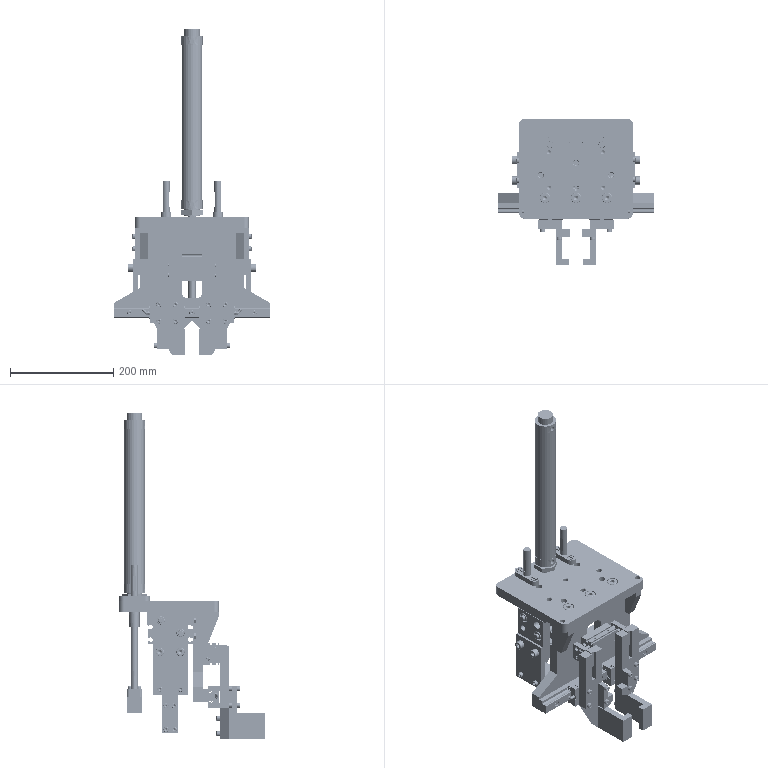Assembly | NX | mm | 90 component files | 90 solids | 2789 faces | box 300 x 282.7 x 629.92 mm | volume 4094625 mm3 | plane 1543 | cone 552 | cylinder 475 | spline 109 | torus 108 | sphere 2 | commonest cylinder face diameters 6 x76 5 x65 10 x55 8 x34 3.5 x28 20 x23 4.2 x18 6.6 x17
Bill of materials:
unnamed part 1 | 2 |  | Flanged post: a flat obround (slot-shaped) flange with a cylindrical post perpendicular to it at the center. A central bore runs down through the post, and there is a counterbored hole near each rounded end of the flange.
unnamed part 2 | 4 |  | Slotted cheese-style screw: a cylindrical head with slightly tapered sides and a straight slot across the top, a short plain neck, and an externally threaded shank.
unnamed part 3 | 2 |  | Rectangular block with a stepped notch along one lower edge. It has several round through holes of different sizes, and two cylindrical pins pass through it, sticking out a long way on one face and a short way on the other.
unnamed part 4 | 2 |  | Angled fitting-like body: a straight cylindrical section with a hex band partway along it, joined by a rounded bend to a shorter angled section. The angled section has a hex collar and a tapered, faceted end.
unnamed part 5 | 12 |  | Socket head cap screw style fastener: a cylindrical head with a hexagonal socket recess on top and a long, fully threaded shank.
unnamed part 6 | 1 |  | Rectangular prismatic block. One long face has two parallel lengthwise grooves with two drilled holes between them. An end face has four large round holes and four edge notches with rounded bottoms, and the side faces have smaller holes.
unnamed part 7 | 2 |  | Slender cylindrical pin or rod with a short reduced-diameter neck (groove) near one end. A possible small flat or surface feature is also visible near that end.
unnamed part 8 | 5 |  | Short socket head cap screw style fastener: a cylindrical head with a hexagonal socket and a threaded shank about one and a half head lengths long.
unnamed part 9 | 2 |  | L-shaped block of constant thickness: a tall rectangular leg and a shorter, wider foot portion with an angled cut at its bottom. Two round through holes are spaced along the tall leg.
unnamed part 10 | 4 |  | Hex head bolt style fastener: a hexagonal head with chamfered corners and a threaded shank running almost to the head.
unnamed part 11 | 2 |  | Thin rectangular plate with four round through holes near the corners: two larger holes at one end and two smaller at the other. There is a shallow rectangular groove or step across one face near the small-hole end.
unnamed part 12 | 2 |  | Bracket of two flat plates joined at a right angle: a solid rectangular top plate and a narrower vertical web, flush with one edge of the top plate, with four round through holes in a 2x2 pattern. It looks T-shaped from one side and L-shaped from the other.
unnamed part 13 | 4 |  | Long socket-head cap screw: a cylindrical head with a hexagonal socket recess on a long, fully threaded slender shank.
unnamed part 14 | 2 |  | Flat bar plate with a straight open-ended slot cut in from one end, a tapered (angled) edge at the opposite end, and a pattern of small through-holes.
unnamed part 15 | 3 |  | Rectangular block with a V-shaped notch cut across one face, leaving two lugs, each with two through-holes.
unnamed part 16 | 2 |  | Rectangular plate with a stepped edge, with two parallel cylindrical rods pressed through it. The rods stick out a short way on one side and a long way on the other. The plate also has extra holes.
unnamed part 17 | 4 |  | Short socket-head-style cap screw with a cylindrical head and a fully threaded shank.
unnamed part 18 | 4 |  | Thin rectangular plate with a large C-shaped cutout on one long edge. The cutout has lobed/notched corners, and the plate carries raised or recessed features, including two small counterbored hex-shaped holes.
unnamed part 19 | 1 |  | Upright rectangular plate on a wider base flange with angled gussets at both sides. It has a central rounded-rectangle through-slot and several hole patterns.
unnamed part 20 | 2 |  | Solid prismatic wedge block: rectangular in two views, with one face tapered at an angle along most of its height.
unnamed part 21 | 2 |  | Rectangular block with a C-shaped channel profile running its full length. The middle body is slightly larger than the end sections, and there are mounting holes on the top and side faces.
unnamed part 22 | 1 |  | Flat rectangular plate with rounded corners, many through-holes of several sizes (some counterbored), and a small rectangular notch on one edge underside.
unnamed part 23 | 4 |  | Socket-head cap screw with a cylindrical head, a hexagonal socket and a fully threaded shank of moderate length.
unnamed part 24 | 2 |  | L-section rectangular bar or block: a thin plate with a short perpendicular foot along one edge, extruded with a constant profile.
unnamed part 25 | 4 |  | Socket head cap screw-like fastener: cylindrical head with hexagonal socket, long fully threaded shank.
unnamed part 26 | 1 |  | Rectangular bar/plate with rounded corners and a symmetric pattern of holes: two larger holes near the ends, a larger central through hole, and four smaller through holes around the center.
unnamed part 27 | 1 |  | Long straight prismatic rail with a constant profile featuring longitudinal grooves on the side faces and a row of five evenly spaced holes along its length.
unnamed part 28 | 4 |  | Socket head cap screw-like fastener with cylindrical head, hexagonal socket and a threaded shank of moderate length.
unnamed part 29 | 1 |  | Slender elongated cylindrical body with end caps, a smaller-diameter rod extending from one end, and a hexagonal flange/collar feature near the rod end.
unnamed part 30 | 4 |  | Cap-screw-like fastener with a plain cylindrical head and a long threaded shank.
unnamed part 31 | 1 |  | Rectangular block with longitudinal grooves along two opposite sides, a shallow large circular recess and multiple small holes on the top face, through holes on the end faces, and semicircular edge notches.
unnamed part 32 | 3 |  | Short socket head cap screw-like fastener: cylindrical head with hexagonal socket and a short threaded shank.
Mates:
1. touch align | Cyl_Fix_Plate 1 face | Cyl_Fix_Vert_Plate 1 face
2. concentric | Cyl_Fix_Vert_Plate 1 edge | Cyl_Fix_Plate 1 edge
3. concentric | V_Block 3 edge | V_Block_Fix_Plate 1 edge
4. concentric | V_Block 3 edge | V_Block_Fix_Plate 1 edge
5. concentric | Reinforce_Rib 1 edge | Cyl_Fix_Vert_Plate 1 edge
6. concentric | Reinforce_Rib 2 edge | Cyl_Fix_Vert_Plate 1 edge
7. concentric | Reinforce_Rib 2 edge | Cyl_Fix_Vert_Plate 1 edge
8. concentric | Reinforce_Rib 1 edge | Cyl_Fix_Vert_Plate 1 edge
9. concentric | Column_Cyl 1 edge | V_Block_Fix_Plate 1 edge
10. concentric | Guide_Rod 1 edge | V_Block_Fix_Plate 1 edge
11. concentric | Guide_Rod 2 edge | V_Block_Fix_Plate 1 edge
12. concentric | Guide_Bush 2 edge | Cyl_Fix_Plate 1 edge
13. concentric | Guide_Bush 2 edge | Cyl_Fix_Plate 1 edge
14. concentric | Guide_Bush 1 edge | Cyl_Fix_Plate 1 edge
15. concentric | Guide_Bush 1 edge | Cyl_Fix_Plate 1 edge
16. concentric | Clamp_Cyl_1 1 edge | Cyl_Fix_Vert_Plate 1 edge
17. concentric | Clamp_Cyl_1 1 edge | Cyl_Fix_Vert_Plate 1 edge
18. concentric | Nylon_Stopper_Block 1 edge | Aux_Gripper_Jaw_Vert_Plate 1 edge
19. concentric | Nylon_Stopper_Block 2 edge | Aux_Gripper_Jaw_Vert_Plate 2 edge
20. concentric | Nylon_Stopper_Block 1 edge | Aux_Gripper_Jaw_Vert_Plate 1 edge
21. concentric | Nylon_Stopper_Block 2 edge | Aux_Gripper_Jaw_Vert_Plate 2 edge
22. fit | Guide_Rod 2 face | Guide_Bush 2 edge
23. fit | Guide_Rod 1 face | Guide_Bush 1 face
24. fit | Aux_Clamp_Cyl_Comp 1 face | Clamp_Cyl_1 1 edge
25. fit | Aux_Clamp_Cyl_Comp 2 face | Clamp_Cyl_1 1 edge
26. fit | Aux_Clamp_Cyl_Comp 2 face | Clamp_Cyl_1 1 edge
27. fit | Aux_Clamp_Cyl_Comp 1 face | Clamp_Cyl_1 1 edge
28. touch align | Guide_Rail_1 1 face | Cyl_Fix_Vert_Plate 1 face
29. touch align | Cyl_Fix_Vert_Plate 1 face | Guide_Rail_1 1 face
30. fix | Cyl_Fix_Plate 1 component
31. align lock | Cyl_Fix_Vert_Plate 1 edge | Guide_Rail_1 1 edge
32. align lock | Clamp_Plate 2 edge | Aux_Gripper_Jaw_Vert_Plate 2 edge
33. align lock | Clamp_Plate 1 edge | Aux_Gripper_Jaw_Vert_Plate 1 edge
34. align lock | Slider_1_Clamp_Plate 4 edge | Slider_2 2 edge
35. align lock | Slider_1_Clamp_Plate 4 edge | Slider_2 2 edge
36. align lock | Slider_1_Clamp_Plate 4 edge | Slider_2 2 edge
37. align lock | Slider_1_Clamp_Plate 1 edge | Slider_2 2 edge
38. align lock | Slider_1_Clamp_Plate 1 edge | Slider_2 2 edge
39. align lock | Slider_2 2 edge | Slider_1_Clamp_Plate 1 edge
40. align lock | Slider_1_Clamp_Plate 3 edge | Slider_2 1 edge
41. align lock | Slider_1_Clamp_Plate 3 edge | Slider_2 1 edge
42. align lock | Slider_2 1 edge | Slider_1_Clamp_Plate 3 edge
43. align lock | Slider_1_Clamp_Plate 2 edge | Slider_2 1 edge
44. align lock | Slider_1_Clamp_Plate 2 edge | Slider_2 1 edge
45. align lock | Slider_2 1 edge | Slider_1_Clamp_Plate 2 edge
46. concentric | Slider_2 2 edge | Aux_Gripper_Jaw_Vert_Plate 2 edge
47. concentric | Slider_2 2 edge | Aux_Gripper_Jaw_Vert_Plate 2 edge
48. concentric | Slider_2 1 edge | Aux_Gripper_Jaw_Vert_Plate 1 edge
49. concentric | Slider_2 1 edge | Aux_Gripper_Jaw_Vert_Plate 1 edge
50. center | Slider_2 2 face | Slider_2 2 face | Guide_Rail_1 1 face
51. touch align | Slider_1_Clamp_Plate 1 face | Guide_Rail_1 1 face
52. center | Slider_2 1 face | Slider_2 1 face | Guide_Rail_1 1 face
53. touch align | Slider_1_Clamp_Plate 3 face | Guide_Rail_1 1 face
54. center | Aux_Gripper_Jaw_Vert_Plate 1 face | Aux_Gripper_Jaw_Vert_Plate 1 face | Aux_Clamp_Cyl_Comp 1 face | Aux_Clamp_Cyl_Comp 1 face
55. center | Aux_Gripper_Jaw_Vert_Plate 2 face | Aux_Gripper_Jaw_Vert_Plate 2 face | Aux_Clamp_Cyl_Comp 2 face | Aux_Clamp_Cyl_Comp 2 face
56. center | Aux_Clamp_Cyl_Comp 1 face | Aux_Clamp_Cyl_Comp 2 face | Clamp_Cyl_1 1 face | Clamp_Cyl_1 1 face
57. concentric | Slider_3 1 edge | Slider_1_Clamp_Plate 3 edge
58. angle | Slider_3 1 face | Slider_1_Clamp_Plate 3 edge
59. concentric | Slider_3 2 edge | Slider_1_Clamp_Plate 1 edge
60. angle | Slider_3 2 face | Slider_1_Clamp_Plate 1 edge
61. concentric | Cyl_Fix_Vert_Plate 1 edge | Cyl_Fix_Plate 1 edge
62. concentric | Clamp_Cyl 1 edge | Cyl_Fix_Plate 1 edge
63. concentric | Clamp_Cyl 1 edge | Cyl_Fix_Plate 1 edge
64. concentric | Gripper_Jaw_Vert_Plate 2 edge | Gripper_Jaw_2 2 edge
65. concentric | Gripper_Jaw_Vert_Plate 1 edge | Gripper_Jaw_2 1 edge
66. concentric | Gripper_Jaw_Vert_Plate 2 edge | Gripper_Jaw_2 2 edge
67. concentric | Gripper_Jaw_2 1 edge | Gripper_Jaw_Vert_Plate 1 edge
68. align lock | Clamp_Cyl 1 face | Clamp_Cyl_Comp 2 face
69. align lock | Clamp_Cyl_Comp 1 face | Clamp_Cyl 1 face
70. concentric | Gripper_Jaw_2 1 edge | Clamp_Cyl_Comp 1 edge
71. concentric | Gripper_Jaw_2 1 edge | Clamp_Cyl_Comp 1 edge
72. concentric | Clamp_Cyl_Comp 2 edge | Gripper_Jaw_2 2 edge
73. concentric | Gripper_Jaw_2 2 edge | Clamp_Cyl_Comp 2 edge
74. concentric | V_Block 2 edge | Gripper_Jaw_Vert_Plate 2 edge
75. concentric | V_Block 1 edge | Gripper_Jaw_Vert_Plate 1 edge
76. align lock | Gripper_Jaw_Vert_Plate 2 edge | V_Block 2 edge
77. align lock | V_Block 1 edge | Gripper_Jaw_Vert_Plate 1 edge
78. center | Clamp_Cyl_Comp 2 face | Clamp_Cyl_Comp 1 face | Clamp_Cyl 1 face | Clamp_Cyl 1 face
79. concentric | M8_Slotted_Bolt 4 edge | Guide_Bush 2 edge
80. concentric | M8_Slotted_Bolt 2 edge | Guide_Bush 2 edge
81. concentric | M8_Slotted_Bolt 3 edge | Guide_Bush 1 edge
82. concentric | M8_Slotted_Bolt 1 edge | Guide_Bush 1 edge
83. concentric | M6x12_Int 3 edge | Guide_Rail_1 1 edge
84. concentric | M6x12_Int 5 edge | Guide_Rail_1 1 edge
85. concentric | M6x12_Int 2 edge | Guide_Rail_1 1 edge
86. concentric | M6x12_Int 4 edge | Guide_Rail_1 1 edge
87. concentric | M6x12_Int 1 edge | Guide_Rail_1 1 edge
88. concentric | M6x20_Int 4 edge | Cyl_Fix_Vert_Plate 1 edge
89. concentric | M6x20_Int 3 edge | Cyl_Fix_Vert_Plate 1 edge
90. concentric | M6x20_Int 2 edge | Cyl_Fix_Vert_Plate 1 edge
91. concentric | M6x20_Int 1 edge | Cyl_Fix_Vert_Plate 1 edge
92. concentric | M6x20_Ext 4 edge | Cyl_Fix_Vert_Plate 1 edge
93. concentric | M6x20_Ext 1 edge | Cyl_Fix_Vert_Plate 1 edge
94. concentric | M6x20_Ext 2 edge | Cyl_Fix_Vert_Plate 1 edge
95. concentric | M6x20_Ext 3 edge | Cyl_Fix_Vert_Plate 1 edge
96. concentric | M10x20_Int 1 edge | Cyl_Fix_Plate 1 edge
97. concentric | M10x20_Int 2 edge | Cyl_Fix_Plate 1 edge
98. concentric | M10x20_Int 3 edge | Cyl_Fix_Plate 1 edge
99. parallel | M10x20_Int 3 face | Cyl_Fix_Plate 1 face
100. parallel | M10x20_Int 1 face | Cyl_Fix_Plate 1 face
101. parallel | M10x20_Int 2 face | Cyl_Fix_Plate 1 face
102. parallel | M6x20_Int 4 face | Cyl_Fix_Vert_Plate 1 face
103. parallel | M6x20_Int 2 face | Cyl_Fix_Vert_Plate 1 face
104. parallel | M6x20_Int 1 face | Cyl_Fix_Vert_Plate 1 face
105. parallel | M6x20_Int 3 face | Cyl_Fix_Vert_Plate 1 face
106. parallel | M6x20_Ext 2 face | Cyl_Fix_Vert_Plate 1 face
107. parallel | M6x20_Ext 3 face | Cyl_Fix_Vert_Plate 1 face
108. parallel | M6x20_Ext 4 face | Cyl_Fix_Vert_Plate 1 face
109. parallel | M6x20_Ext 1 face | Cyl_Fix_Vert_Plate 1 face
110. parallel | M6x12_Int 5 face | Cyl_Fix_Vert_Plate 1 face
111. parallel | M6x12_Int 3 face | Cyl_Fix_Vert_Plate 1 face
112. parallel | M6x12_Int 2 face | Cyl_Fix_Vert_Plate 1 face
113. parallel | M6x12_Int 4 face | Cyl_Fix_Vert_Plate 1 face
114. parallel | M6x12_Int 1 face | Cyl_Fix_Vert_Plate 1 face
115. parallel | M8_Slotted_Bolt 4 edge | Guide_Bush 2 edge
116. parallel | M8_Slotted_Bolt 2 edge | Guide_Bush 2 edge
117. parallel | M8_Slotted_Bolt 1 edge | Guide_Bush 1 edge
118. parallel | M8_Slotted_Bolt 3 edge | Guide_Bush 1 edge
119. concentric | M5_Hex_Bolt 2 edge | Nylon_Stopper_Block 2 edge
120. concentric | M5_Hex_Bolt 4 edge | Nylon_Stopper_Block 2 edge
121. concentric | M5_Hex_Bolt 3 edge | Nylon_Stopper_Block 1 edge
122. concentric | M5_Hex_Bolt 1 edge | Nylon_Stopper_Block 1 edge
123. concentric | M5x25_Hex_Bolt 3 edge | Aux_Gripper_Jaw_Vert_Plate 2 edge
124. concentric | M5x25_Hex_Bolt 4 edge | Aux_Gripper_Jaw_Vert_Plate 2 edge
125. concentric | M5x25_Hex_Bolt 2 edge | Aux_Gripper_Jaw_Vert_Plate 1 edge
126. concentric | M5x25_Hex_Bolt 1 edge | Aux_Gripper_Jaw_Vert_Plate 1 edge
127. concentric | M5x30_Hex_Bolt 4 edge | Aux_Gripper_Jaw_Vert_Plate 2 edge
128. concentric | M5x30_Hex_Bolt 3 edge | Aux_Gripper_Jaw_Vert_Plate 2 edge
129. concentric | M5x30_Hex_Bolt 2 edge | Aux_Gripper_Jaw_Vert_Plate 1 edge
130. concentric | M5x30_Hex_Bolt 1 edge | Aux_Gripper_Jaw_Vert_Plate 1 edge
131. parallel | M5x30_Hex_Bolt 3 face | Aux_Gripper_Jaw_Vert_Plate 2 face
132. parallel | M5x30_Hex_Bolt 4 face | Aux_Gripper_Jaw_Vert_Plate 2 face
133. parallel | M5x30_Hex_Bolt 1 face | Aux_Gripper_Jaw_Vert_Plate 1 face
134. parallel | M5x30_Hex_Bolt 2 face | Aux_Gripper_Jaw_Vert_Plate 1 face
135. parallel | M5x25_Hex_Bolt 4 face | Aux_Gripper_Jaw_Vert_Plate 2 face
136. parallel | M5x25_Hex_Bolt 3 face | Aux_Gripper_Jaw_Vert_Plate 2 face
137. parallel | M5_Hex_Bolt 4 face | Clamp_Plate 2 face
138. parallel | M5_Hex_Bolt 2 face | Clamp_Plate 2 face
139. parallel | M5_Hex_Bolt 1 face | Clamp_Plate 1 face
140. parallel | M5_Hex_Bolt 3 face | Clamp_Plate 1 face
141. parallel | M5x25_Hex_Bolt 1 face | Clamp_Plate 1 face
142. parallel | M5x25_Hex_Bolt 2 face | Clamp_Plate 1 face
143. concentric | M6x20_Hex_Bolt 1 edge | Gripper_Jaw_2 2 edge
144. concentric | M6x20_Hex_Bolt 4 edge | Gripper_Jaw_2 2 edge
145. concentric | M6x20_Hex_Bolt 2 edge | Gripper_Jaw_2 1 edge
146. concentric | M6x20_Hex_Bolt 3 edge | Gripper_Jaw_2 1 edge
147. parallel | M6x20_Hex_Bolt 3 face | Gripper_Jaw_2 1 face
148. parallel | M6x20_Hex_Bolt 2 face | Gripper_Jaw_2 1 face
149. parallel | M6x20_Hex_Bolt 1 face | Gripper_Jaw_2 2 face
150. parallel | M6x20_Hex_Bolt 4 face | Gripper_Jaw_2 2 face
151. concentric | M8x24_Hex_Bolt 1 edge | Gripper_Jaw_2 2 edge
152. concentric | M8x24_Hex_Bolt 4 edge | Gripper_Jaw_2 2 edge
153. concentric | M8x24_Hex_Bolt 3 edge | Gripper_Jaw_2 1 edge
154. concentric | M8x24_Hex_Bolt 2 edge | Gripper_Jaw_2 1 edge
155. concentric | M6x12_Hex_Bolt 11 edge | Gripper_Jaw_Vert_Plate 2 edge
156. concentric | M6x12_Hex_Bolt 10 edge | Gripper_Jaw_Vert_Plate 2 edge
157. concentric | M6x12_Hex_Bolt 12 edge | Gripper_Jaw_Vert_Plate 2 edge
158. concentric | M6x12_Hex_Bolt 9 edge | Gripper_Jaw_Vert_Plate 2 edge
159. parallel | M6x12_Hex_Bolt 12 face | Gripper_Jaw_Vert_Plate 2 face
160. parallel | M6x12_Hex_Bolt 9 face | Gripper_Jaw_Vert_Plate 2 face
161. parallel | M6x12_Hex_Bolt 10 face | Gripper_Jaw_Vert_Plate 2 face
162. parallel | M6x12_Hex_Bolt 11 face | Gripper_Jaw_Vert_Plate 2 face
163. concentric | M6x12_Hex_Bolt 7 edge | Gripper_Jaw_Vert_Plate 1 edge
164. concentric | M6x12_Hex_Bolt 8 edge | Gripper_Jaw_Vert_Plate 1 edge
165. concentric | M6x12_Hex_Bolt 3 edge | Gripper_Jaw_Vert_Plate 1 edge
166. concentric | M6x12_Hex_Bolt 4 edge | Gripper_Jaw_Vert_Plate 1 edge
167. parallel | M6x12_Hex_Bolt 3 face | Gripper_Jaw_Vert_Plate 1 face
168. parallel | M6x12_Hex_Bolt 4 face | Gripper_Jaw_Vert_Plate 1 face
169. parallel | M6x12_Hex_Bolt 7 face | Gripper_Jaw_Vert_Plate 1 face
170. parallel | M6x12_Hex_Bolt 8 face | Gripper_Jaw_Vert_Plate 1 face
171. concentric | M6x12_Hex_Bolt 1 edge | V_Block_Fix_Plate 1 edge
172. concentric | M6x12_Hex_Bolt 5 edge | V_Block_Fix_Plate 1 edge
173. concentric | M6x12_Hex_Bolt 6 edge | V_Block_Fix_Plate 1 edge
174. concentric | M6x12_Hex_Bolt 2 edge | V_Block_Fix_Plate 1 edge
175. parallel | M6x12_Hex_Bolt 2 face | V_Block_Fix_Plate 1 face
176. parallel | M6x12_Hex_Bolt 6 face | V_Block_Fix_Plate 1 face
177. parallel | M6x12_Hex_Bolt 5 face | V_Block_Fix_Plate 1 face
178. parallel | M6x12_Hex_Bolt 1 face | V_Block_Fix_Plate 1 face